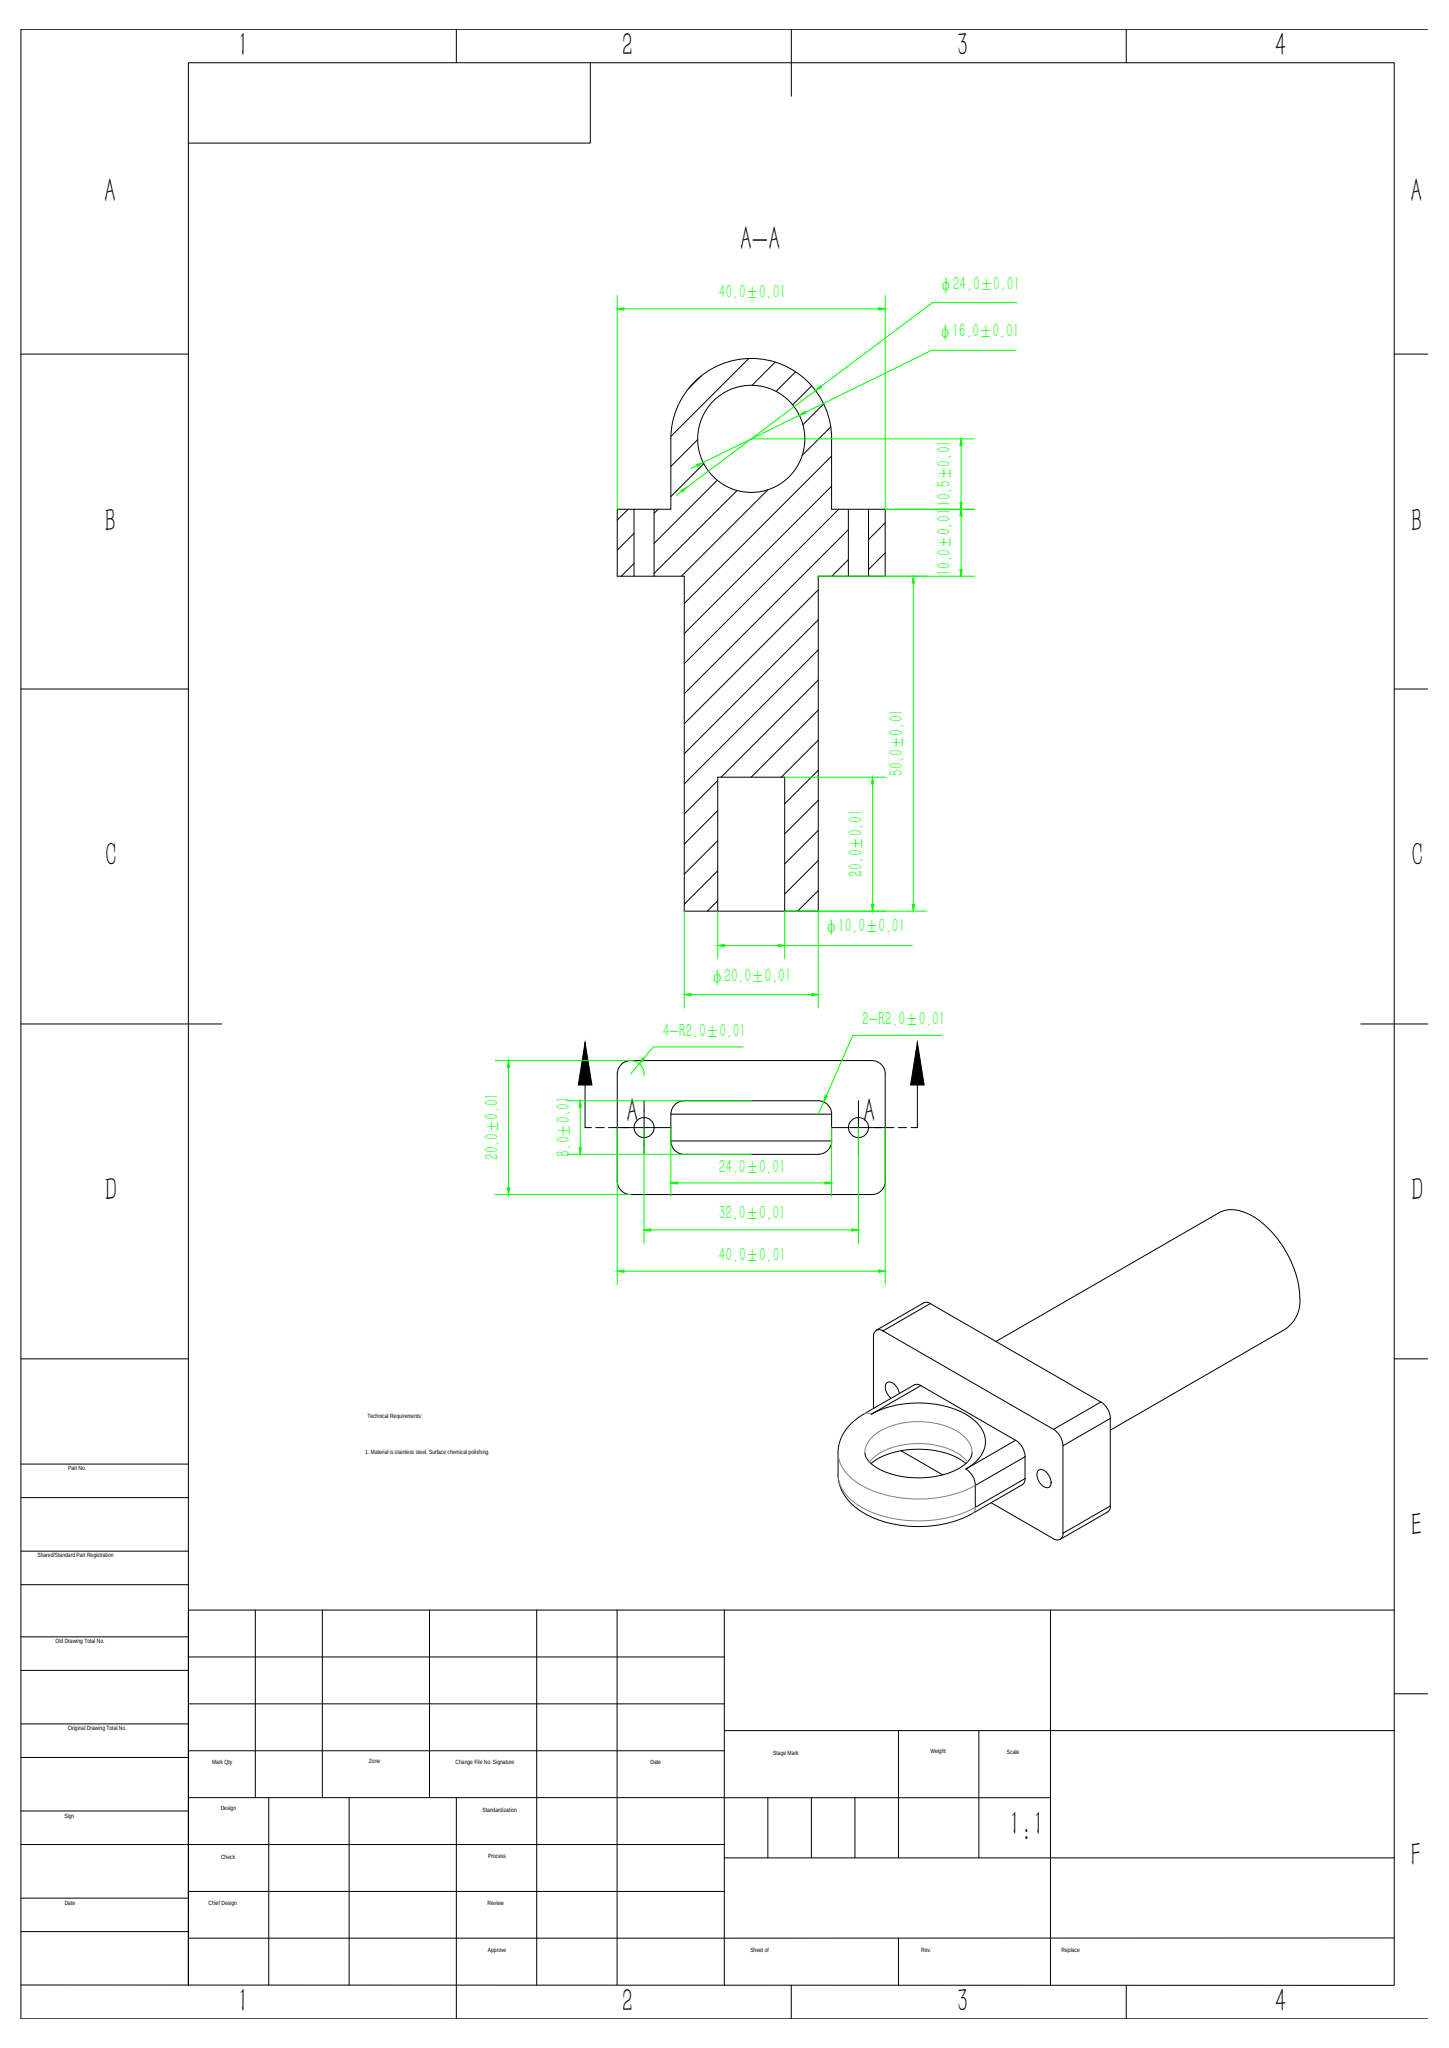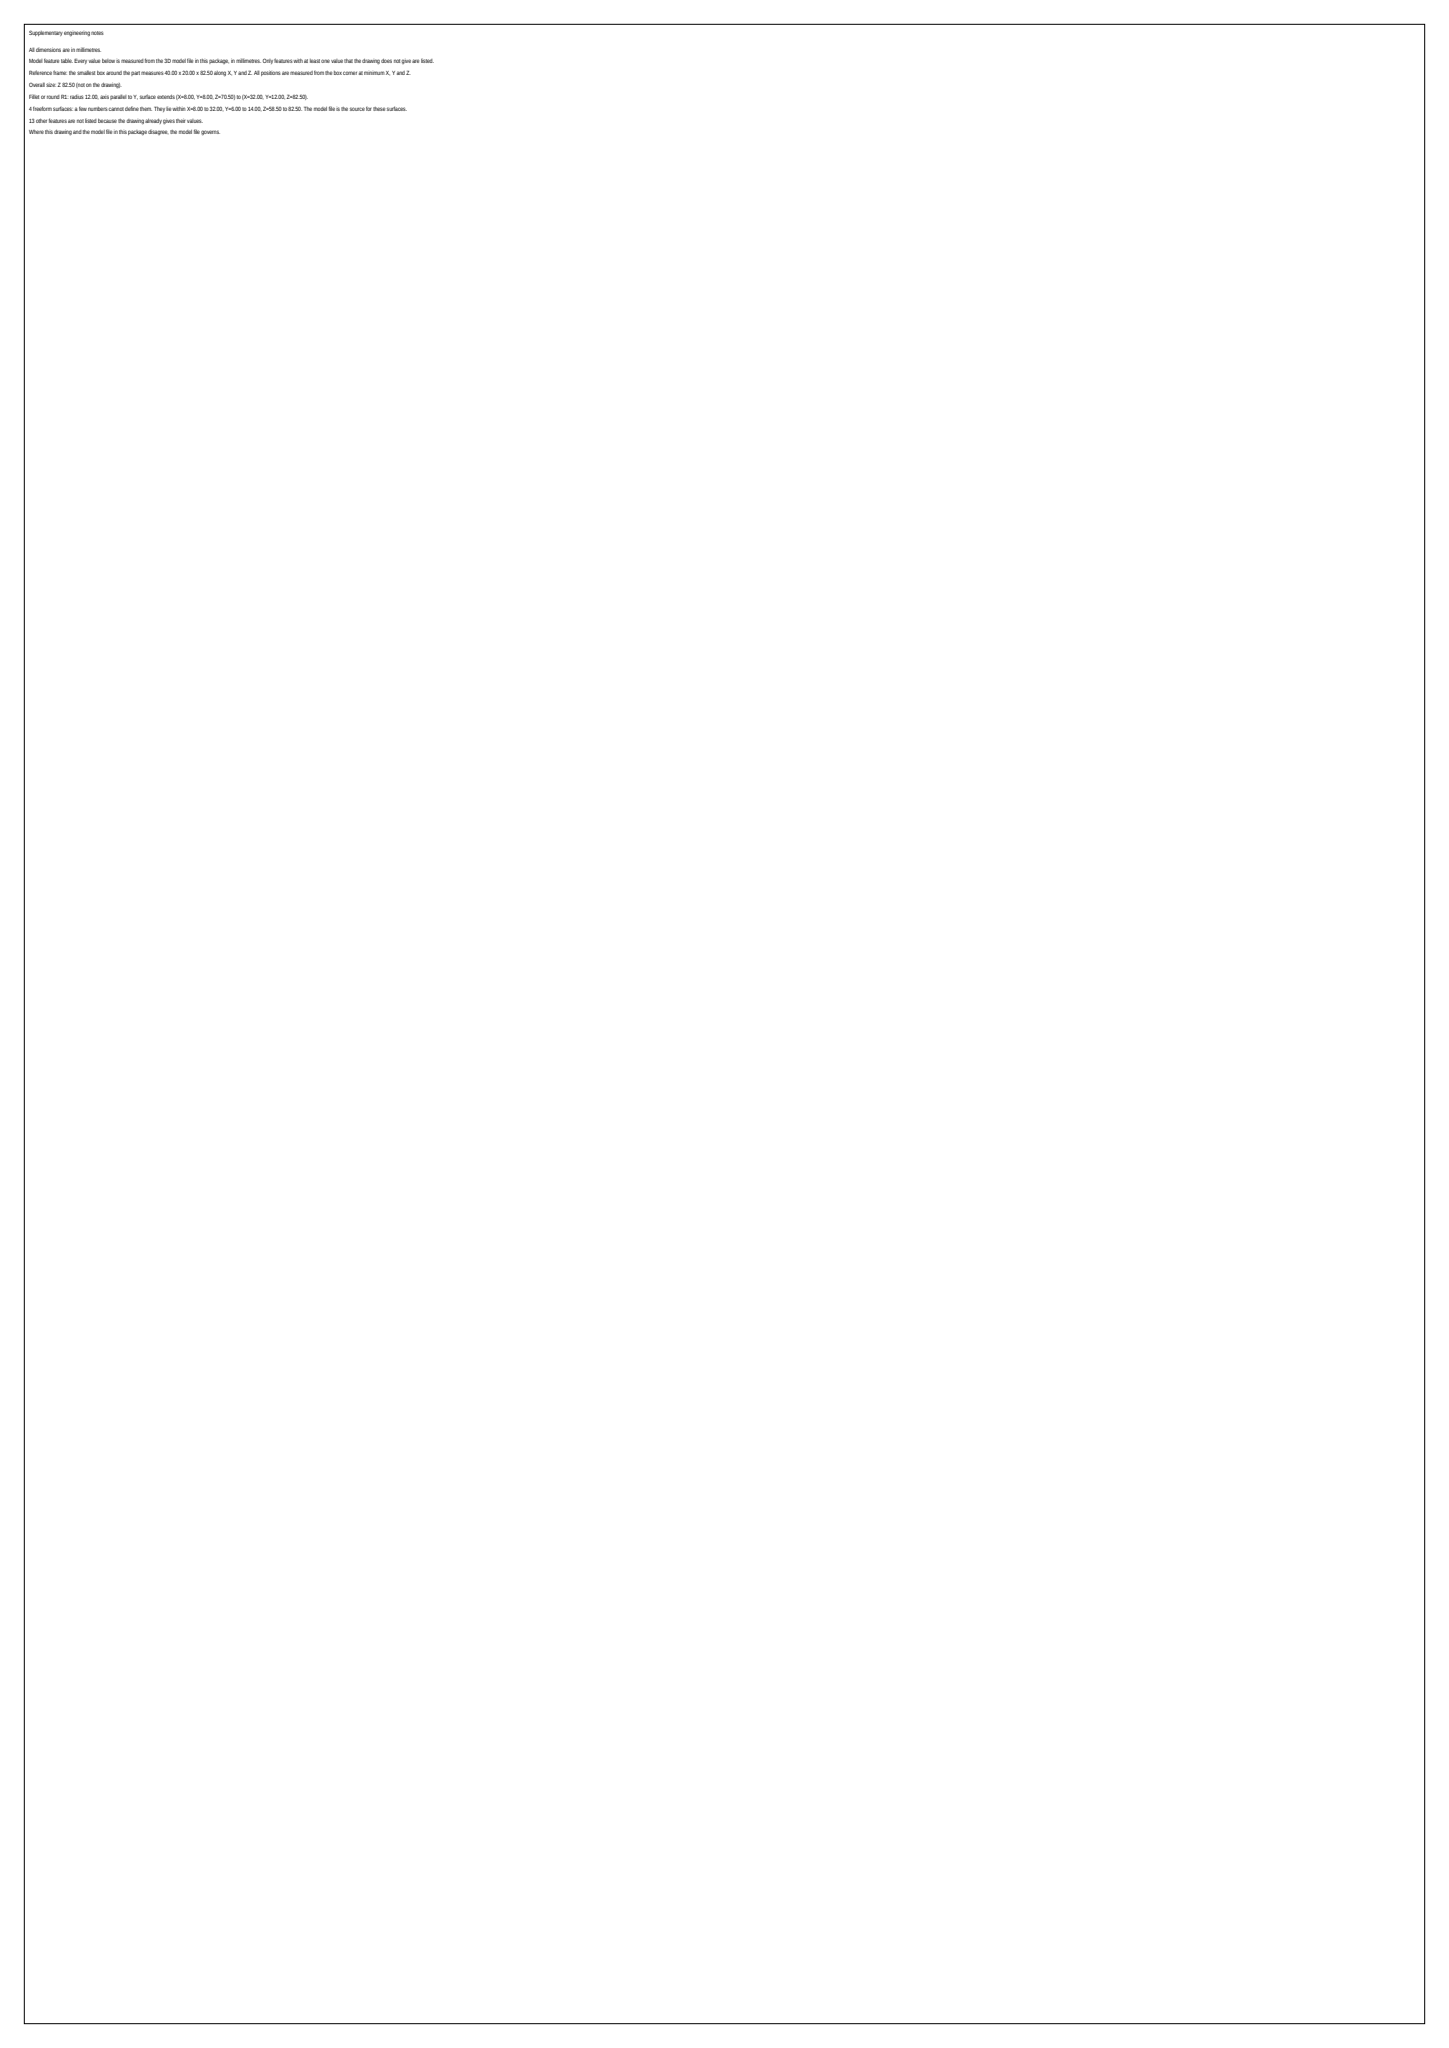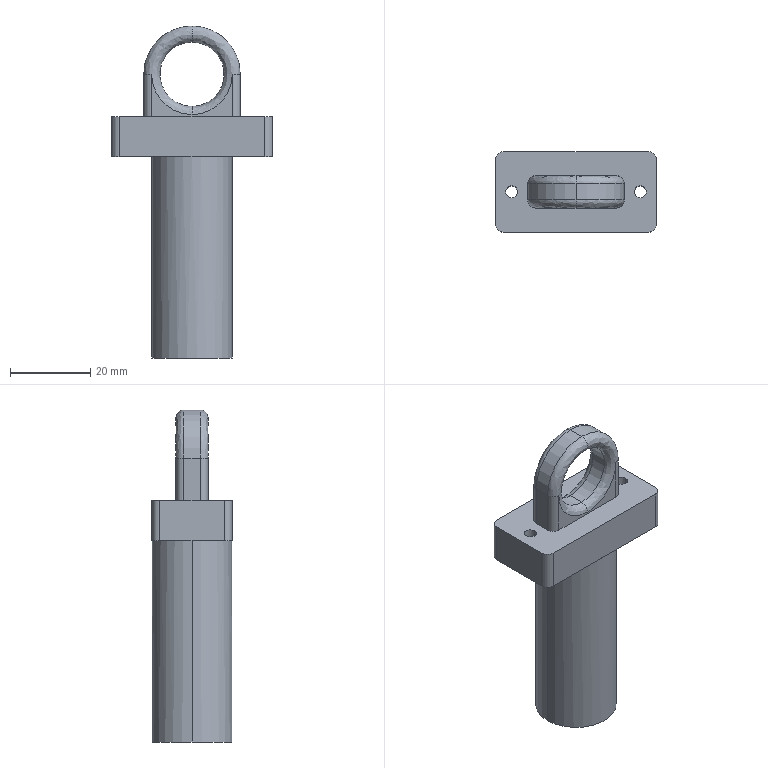Part | SolidWorks | mm | material stainless steel | 1 solid | 37 faces | box 40 x 20 x 82.5 mm | volume 23989 mm3 | cylinder 20 | plane 13 | spline 4 | commonest cylinder face diameters 4 x8 3 x4 20 x2 10 x2 24 x2 16 x2